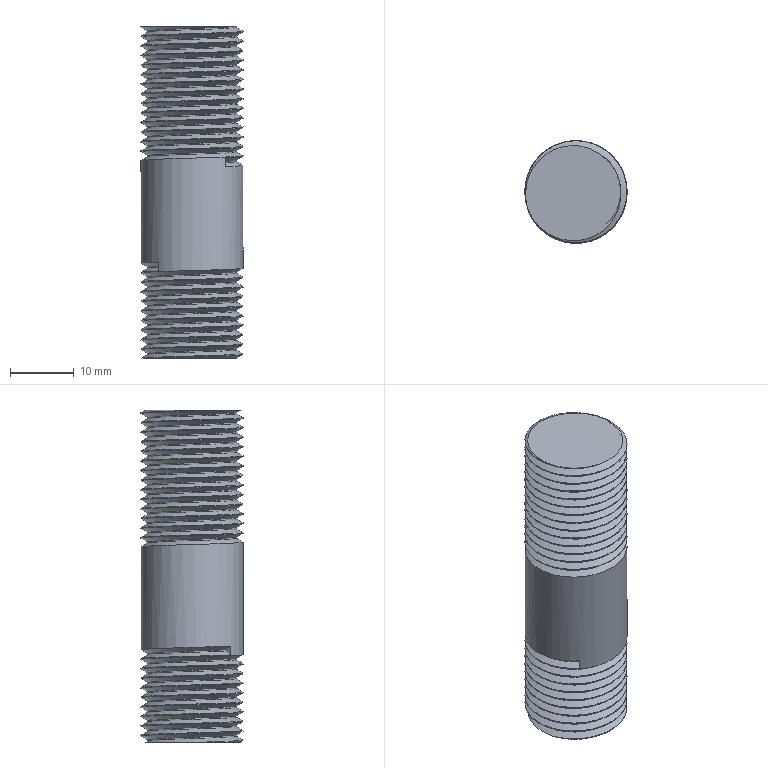Component | NX | 09__STUD_M16X1_5__2 | 1 solid | 34 faces | volume 9559 mm3 | cylinder 26 | plane 4 | spline 4 | commonest cylinder face diameters 16 x24 14 x2